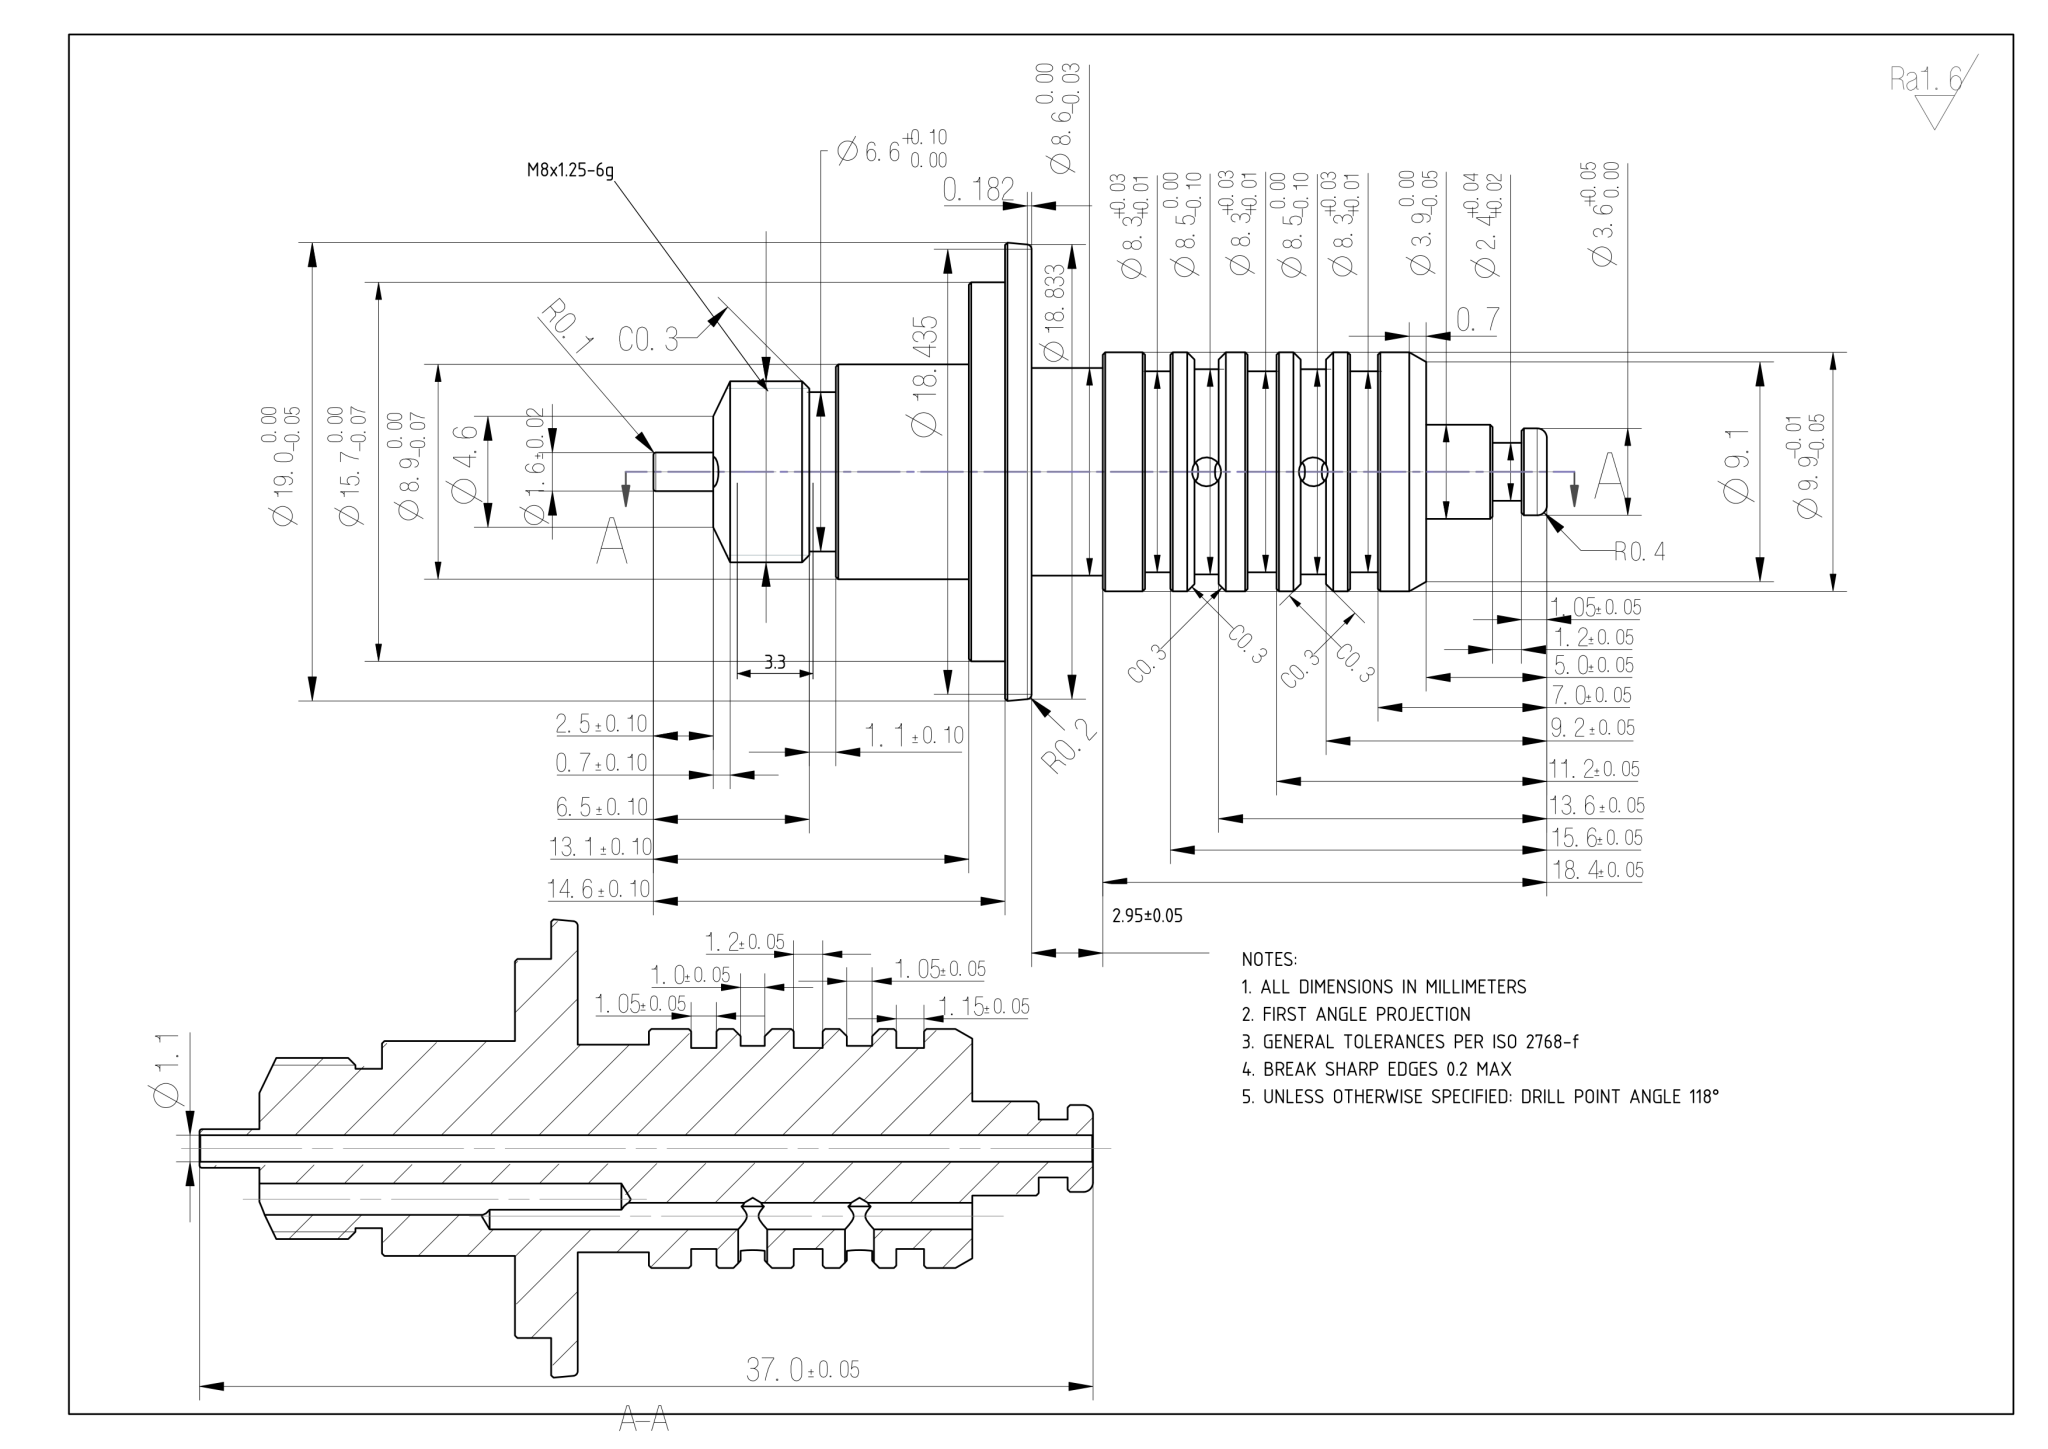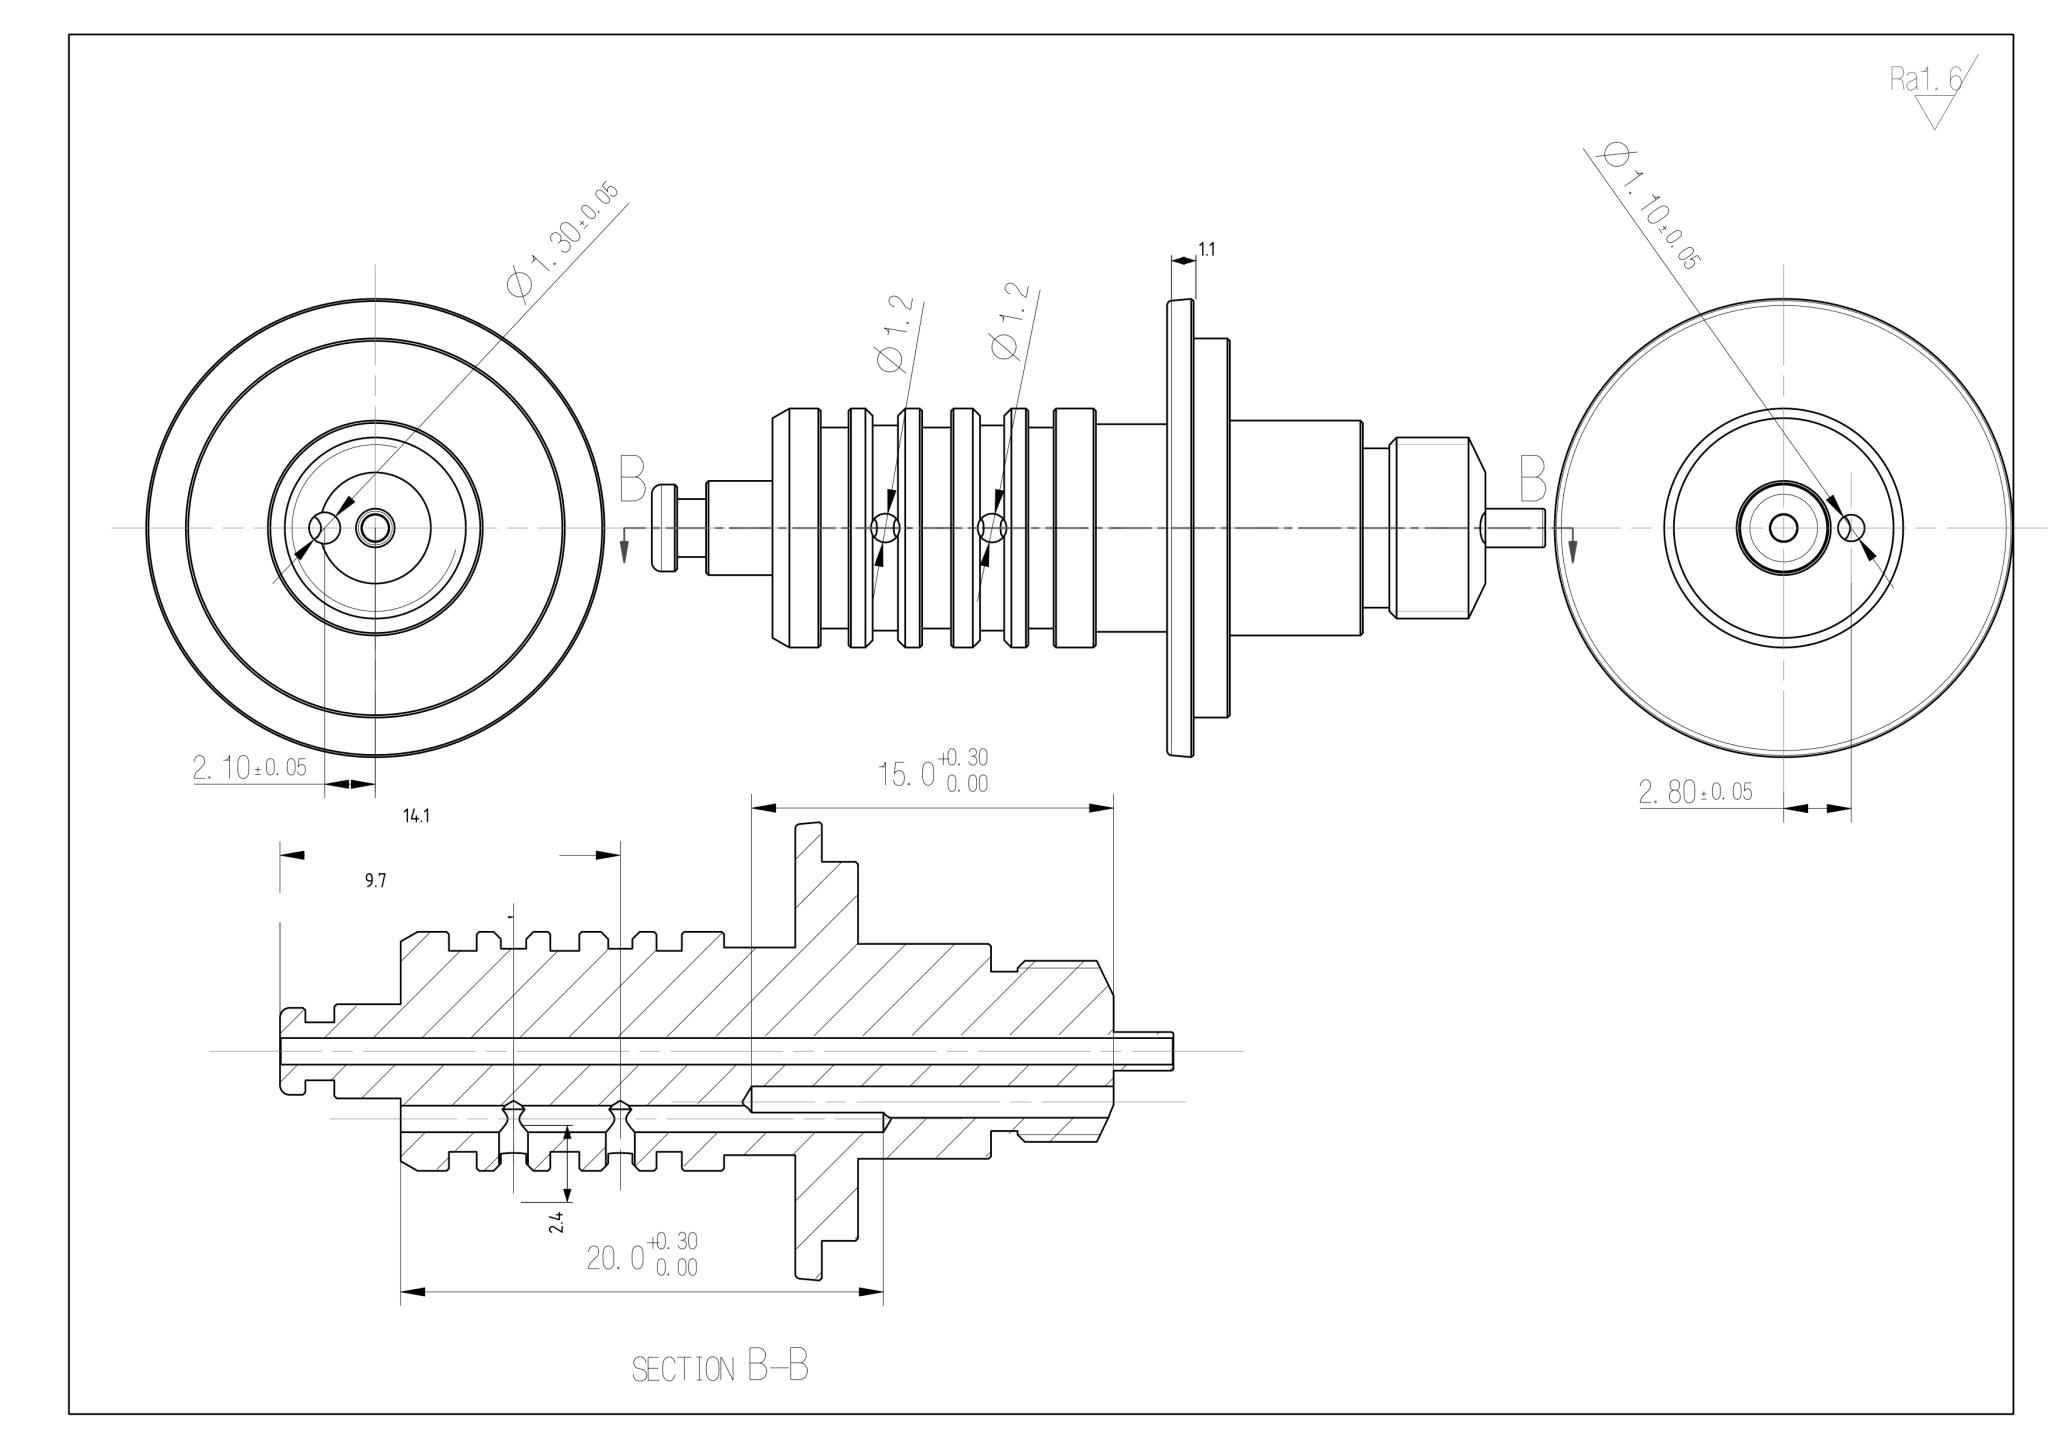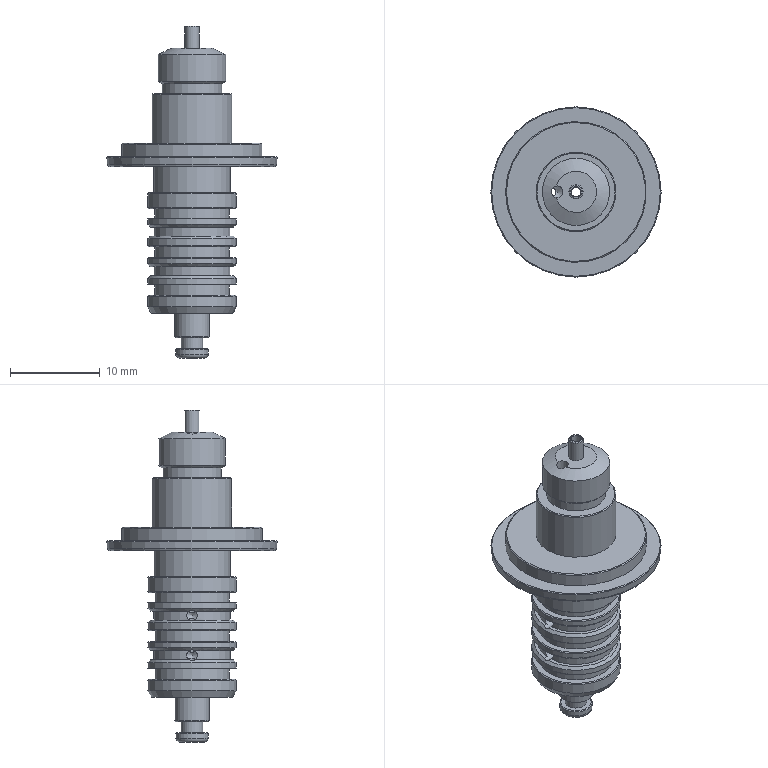Part | NX | mm | 1 solid | 78 faces | box 18.98 x 18.98 x 37.02 mm | volume 2195 mm3 | cylinder 27 | cone 26 | plane 22 | torus 3 | commonest cylinder face diameters 9.9 x6 1.1 x4 8.325 x3 8.5 x2 1.2 x2 1.6 x1 7.5 x1 6.6 x1